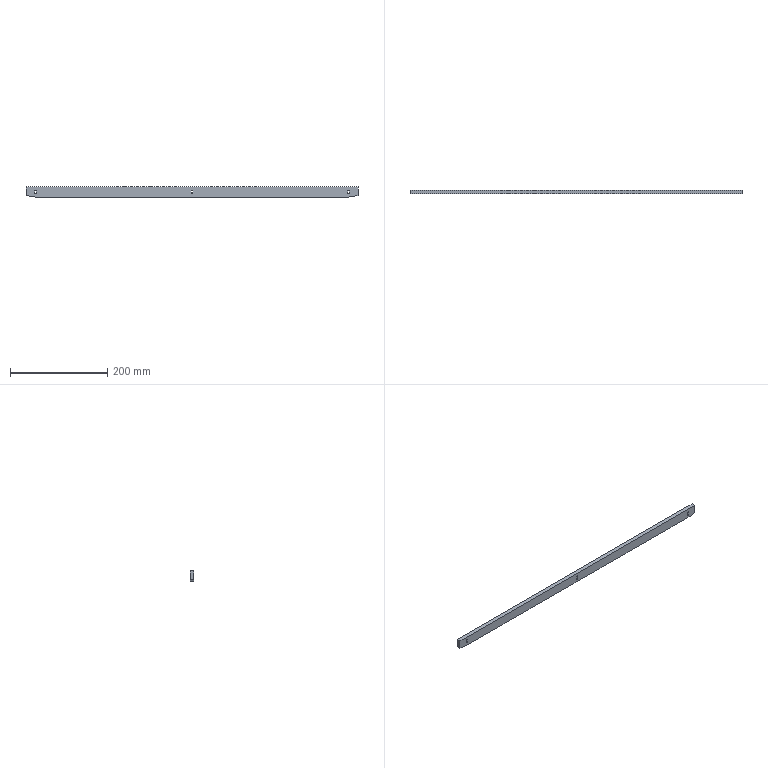Component | SolidWorks | SL010-RightStreamline-1-1_SL010-LXFB-010202-003-1-1 | 1 solid | 20 faces | box 683 x 8 x 21 mm | volume 113687 mm3 | plane 14 | cylinder 6 | commonest cylinder face diameters 3.2 x6 | material S45C
build123d program:
from build123d import *

# Parameters (mm, degrees)
SKETCH1_W           = 683
SKETCH1_H           = 21
BOSS_EXTRUDE1_DEPTH = 8
CUT_EXTRUDE1_DEPTH  = 342.755
CHAMFER1_SIZE       = 3
CHAMFER1_SIZE2      = 20
CHAMFER2_SIZE       = 20
CHAMFER2_SIZE2      = 3


with BuildPart() as part:
    # Sketch1 → Boss-Extrude1 (new body)
    with BuildSketch(Plane.XY):
        Rectangle(SKETCH1_W, SKETCH1_H)
    extrude(amount=BOSS_EXTRUDE1_DEPTH)

    # Sketch2 → Cut-Extrude1 (cut, through all)
    with BuildSketch(Plane.XY.offset(8)):
        with BuildLine():
            Line((-319.9, 2.5), (-319.9, -2.5))
            ThreePointArc((-319.9, -2.5), (-321.5, -4.1), (-323.1, -2.5))
            Line((-323.1, -2.5), (-323.1, 2.5))
            ThreePointArc((-323.1, 2.5), (-321.5, 4.1), (-319.9, 2.5))
        make_face()
        with BuildLine():
            Line((1.6, 2.5), (1.6, -2.5))
            ThreePointArc((1.6, -2.5), (0, -4.1), (-1.6, -2.5))
            Line((-1.6, -2.5), (-1.6, 2.5))
            ThreePointArc((-1.6, 2.5), (0, 4.1), (1.6, 2.5))
        make_face()
        with BuildLine():
            Line((323.1, 2.5), (323.1, -2.5))
            ThreePointArc((323.1, -2.5), (321.5, -4.1), (319.9, -2.5))
            Line((319.9, -2.5), (319.9, 2.5))
            ThreePointArc((319.9, 2.5), (321.5, 4.1), (323.1, 2.5))
        make_face()
    extrude(amount=-CUT_EXTRUDE1_DEPTH, mode=Mode.SUBTRACT)

    # Chamfer1
    chamfer1_edges = [part.edges().sort_by_distance(p)[0] for p in [
        (341.5, 10.5, 4),
    ]]
    chamfer1_side = [part.faces().sort_by_distance(p)[0] for p in [
        (341.5, 0, 4),
    ]]
    chamfer(chamfer1_edges, length=CHAMFER1_SIZE, length2=CHAMFER1_SIZE2, reference=chamfer1_side[0])

    # Chamfer2
    chamfer2_edges = [part.edges().sort_by_distance(p)[0] for p in [
        (-341.5, 10.5, 4),
    ]]
    chamfer2_side = [part.faces().sort_by_distance(p)[0] for p in [
        (-10, 10.5, 4),
    ]]
    chamfer(chamfer2_edges, length=CHAMFER2_SIZE, length2=CHAMFER2_SIZE2, reference=chamfer2_side[0])


solid = part.part

# Placed as in the assembly
solid = solid.moved(Location((633.5, -109.904, -326.535), (-90, 0, 0)))
STEP:
#1=CARTESIAN_POINT('',(38.386,-4.327,-12.442));
#2=VERTEX_POINT('',#1);
#3=CARTESIAN_POINT('',(38.386,-4.327,-13.151));
#4=VERTEX_POINT('',#3);
#5=CARTESIAN_POINT('',(38.386,-4.327,-13.269));
#6=DIRECTION('',(-0.,0.,-1.));
#7=VECTOR('',#6,39.37);
#8=LINE('',#5,#7);
#9=EDGE_CURVE('',#2,#4,#8,.T.);
#10=ORIENTED_EDGE('',*,*,#9,.T.);
#11=CARTESIAN_POINT('',(38.386,-4.012,-13.151));
#12=VERTEX_POINT('',#11);
#13=CARTESIAN_POINT('',(38.386,-4.012,-13.151));
#14=DIRECTION('',(-0.,1.,-0.));
#15=VECTOR('',#14,39.37);
#16=LINE('',#13,#15);
#17=EDGE_CURVE('',#4,#12,#16,.T.);
#18=ORIENTED_EDGE('',*,*,#17,.T.);
#19=CARTESIAN_POINT('',(38.386,-4.012,-12.442));
#20=VERTEX_POINT('',#19);
#21=CARTESIAN_POINT('',(38.386,-4.012,-13.269));
#22=DIRECTION('',(-0.,0.,-1.));
#23=VECTOR('',#22,39.37);
#24=LINE('',#21,#23);
#25=EDGE_CURVE('',#20,#12,#24,.T.);
#26=ORIENTED_EDGE('',*,*,#25,.F.);
#27=CARTESIAN_POINT('',(38.386,-4.012,-12.442));
#28=DIRECTION('',(0.,-1.,0.));
#29=VECTOR('',#28,39.37);
#30=LINE('',#27,#29);
#31=EDGE_CURVE('',#20,#2,#30,.T.);
#32=ORIENTED_EDGE('',*,*,#31,.T.);
#33=EDGE_LOOP('',(#10,#18,#26,#32));
#34=FACE_OUTER_BOUND('',#33,.T.);
#35=CARTESIAN_POINT('',(38.386,-4.012,-13.269));
#36=DIRECTION('',(-1.,-0.,-0.));
#37=DIRECTION('',(-0.,1.,-0.));
#38=AXIS2_PLACEMENT_3D('',#35,#36,#37);
#39=PLANE('',#38);
#40=ADVANCED_FACE('',(#34),#39,.F.);
#41=CARTESIAN_POINT('',(37.598,-4.327,-13.269));
#42=VERTEX_POINT('',#41);
#43=CARTESIAN_POINT('',(12.283,-4.327,-13.269));
#44=VERTEX_POINT('',#43);
#45=CARTESIAN_POINT('',(11.496,-4.327,-13.269));
#46=DIRECTION('',(-1.,0.,-0.));
#47=VECTOR('',#46,39.37);
#48=LINE('',#45,#47);
#49=EDGE_CURVE('',#42,#44,#48,.T.);
#50=ORIENTED_EDGE('',*,*,#49,.T.);
#51=CARTESIAN_POINT('',(12.283,-4.012,-13.269));
#52=VERTEX_POINT('',#51);
#53=CARTESIAN_POINT('',(12.283,-4.012,-13.269));
#54=DIRECTION('',(-0.,1.,-0.));
#55=VECTOR('',#54,39.37);
#56=LINE('',#53,#55);
#57=EDGE_CURVE('',#44,#52,#56,.T.);
#58=ORIENTED_EDGE('',*,*,#57,.T.);
#59=CARTESIAN_POINT('',(37.598,-4.012,-13.269));
#60=VERTEX_POINT('',#59);
#61=CARTESIAN_POINT('',(11.496,-4.012,-13.269));
#62=DIRECTION('',(-1.,0.,-0.));
#63=VECTOR('',#62,39.37);
#64=LINE('',#61,#63);
#65=EDGE_CURVE('',#60,#52,#64,.T.);
#66=ORIENTED_EDGE('',*,*,#65,.F.);
#67=CARTESIAN_POINT('',(37.598,-4.012,-13.269));
#68=DIRECTION('',(0.,-1.,0.));
#69=VECTOR('',#68,39.37);
#70=LINE('',#67,#69);
#71=EDGE_CURVE('',#60,#42,#70,.T.);
#72=ORIENTED_EDGE('',*,*,#71,.T.);
#73=EDGE_LOOP('',(#50,#58,#66,#72));
#74=FACE_OUTER_BOUND('',#73,.T.);
#75=CARTESIAN_POINT('',(11.496,-4.012,-13.269));
#76=DIRECTION('',(0.,0.,1.));
#77=DIRECTION('',(0.,-1.,0.));
#78=AXIS2_PLACEMENT_3D('',#75,#76,#77);
#79=PLANE('',#78);
#80=ADVANCED_FACE('',(#74),#79,.F.);
#81=CARTESIAN_POINT('',(11.496,-4.012,-13.151));
#82=VERTEX_POINT('',#81);
#83=CARTESIAN_POINT('',(11.496,-4.012,-12.442));
#84=VERTEX_POINT('',#83);
#85=CARTESIAN_POINT('',(11.496,-4.012,-13.269));
#86=DIRECTION('',(0.,-0.,1.));
#87=VECTOR('',#86,39.37);
#88=LINE('',#85,#87);
#89=EDGE_CURVE('',#82,#84,#88,.T.);
#90=ORIENTED_EDGE('',*,*,#89,.F.);
#91=CARTESIAN_POINT('',(11.496,-4.327,-13.151));
#92=VERTEX_POINT('',#91);
#93=CARTESIAN_POINT('',(11.496,-4.012,-13.151));
#94=DIRECTION('',(0.,-1.,0.));
#95=VECTOR('',#94,39.37);
#96=LINE('',#93,#95);
#97=EDGE_CURVE('',#82,#92,#96,.T.);
#98=ORIENTED_EDGE('',*,*,#97,.T.);
#99=CARTESIAN_POINT('',(11.496,-4.327,-12.442));
#100=VERTEX_POINT('',#99);
#101=CARTESIAN_POINT('',(11.496,-4.327,-13.269));
#102=DIRECTION('',(0.,-0.,1.));
#103=VECTOR('',#102,39.37);
#104=LINE('',#101,#103);
#105=EDGE_CURVE('',#92,#100,#104,.T.);
#106=ORIENTED_EDGE('',*,*,#105,.T.);
#107=CARTESIAN_POINT('',(11.496,-4.012,-12.442));
#108=DIRECTION('',(0.,-1.,0.));
#109=VECTOR('',#108,39.37);
#110=LINE('',#107,#109);
#111=EDGE_CURVE('',#84,#100,#110,.T.);
#112=ORIENTED_EDGE('',*,*,#111,.F.);
#113=EDGE_LOOP('',(#90,#98,#106,#112));
#114=FACE_OUTER_BOUND('',#113,.T.);
#115=CARTESIAN_POINT('',(11.496,-4.012,-13.269));
#116=DIRECTION('',(1.,0.,0.));
#117=DIRECTION('',(0.,-1.,0.));
#118=AXIS2_PLACEMENT_3D('',#115,#116,#117);
#119=PLANE('',#118);
#120=ADVANCED_FACE('',(#114),#119,.F.);
#121=CARTESIAN_POINT('',(11.496,-4.327,-12.442));
#122=DIRECTION('',(1.,-0.,0.));
#123=VECTOR('',#122,39.37);
#124=LINE('',#121,#123);
#125=EDGE_CURVE('',#100,#2,#124,.T.);
#126=ORIENTED_EDGE('',*,*,#125,.T.);
#127=ORIENTED_EDGE('',*,*,#31,.F.);
#128=CARTESIAN_POINT('',(11.496,-4.012,-12.442));
#129=DIRECTION('',(1.,-0.,0.));
#130=VECTOR('',#129,39.37);
#131=LINE('',#128,#130);
#132=EDGE_CURVE('',#84,#20,#131,.T.);
#133=ORIENTED_EDGE('',*,*,#132,.F.);
#134=ORIENTED_EDGE('',*,*,#111,.T.);
#135=EDGE_LOOP('',(#126,#127,#133,#134));
#136=FACE_OUTER_BOUND('',#135,.T.);
#137=CARTESIAN_POINT('',(11.496,-4.012,-12.442));
#138=DIRECTION('',(-0.,-0.,-1.));
#139=DIRECTION('',(-0.,1.,-0.));
#140=AXIS2_PLACEMENT_3D('',#137,#138,#139);
#141=PLANE('',#140);
#142=ADVANCED_FACE('',(#136),#141,.F.);
#143=CARTESIAN_POINT('',(37.661,-4.012,-12.954));
#144=VERTEX_POINT('',#143);
#145=CARTESIAN_POINT('',(37.535,-4.012,-12.954));
#146=VERTEX_POINT('',#145);
#147=CARTESIAN_POINT('',(37.598,-4.012,-12.954));
#148=DIRECTION('',(-0.,1.,-0.));
#149=DIRECTION('',(1.,0.,0.));
#150=AXIS2_PLACEMENT_3D('',#147,#148,#149);
#151=CIRCLE('',#150,0.06299);
#152=EDGE_CURVE('',#144,#146,#151,.T.);
#153=ORIENTED_EDGE('',*,*,#152,.F.);
#154=CARTESIAN_POINT('',(37.661,-4.012,-12.757));
#155=VERTEX_POINT('',#154);
#156=CARTESIAN_POINT('',(37.661,-4.012,-12.954));
#157=DIRECTION('',(-0.,0.,-1.));
#158=VECTOR('',#157,39.37);
#159=LINE('',#156,#158);
#160=EDGE_CURVE('',#155,#144,#159,.T.);
#161=ORIENTED_EDGE('',*,*,#160,.F.);
#162=CARTESIAN_POINT('',(37.535,-4.012,-12.757));
#163=VERTEX_POINT('',#162);
#164=CARTESIAN_POINT('',(37.598,-4.012,-12.757));
#165=DIRECTION('',(-0.,1.,-0.));
#166=DIRECTION('',(1.,0.,0.));
#167=AXIS2_PLACEMENT_3D('',#164,#165,#166);
#168=CIRCLE('',#167,0.06299);
#169=EDGE_CURVE('',#163,#155,#168,.T.);
#170=ORIENTED_EDGE('',*,*,#169,.F.);
#171=CARTESIAN_POINT('',(37.535,-4.012,-12.954));
#172=DIRECTION('',(0.,-0.,1.));
#173=VECTOR('',#172,39.37);
#174=LINE('',#171,#173);
#175=EDGE_CURVE('',#146,#163,#174,.T.);
#176=ORIENTED_EDGE('',*,*,#175,.F.);
#177=EDGE_LOOP('',(#153,#161,#170,#176));
#178=FACE_BOUND('',#177,.T.);
#179=CARTESIAN_POINT('',(25.004,-4.012,-12.954));
#180=VERTEX_POINT('',#179);
#181=CARTESIAN_POINT('',(24.878,-4.012,-12.954));
#182=VERTEX_POINT('',#181);
#183=CARTESIAN_POINT('',(24.941,-4.012,-12.954));
#184=DIRECTION('',(-0.,1.,-0.));
#185=DIRECTION('',(1.,0.,0.));
#186=AXIS2_PLACEMENT_3D('',#183,#184,#185);
#187=CIRCLE('',#186,0.06299);
#188=EDGE_CURVE('',#180,#182,#187,.T.);
#189=ORIENTED_EDGE('',*,*,#188,.F.);
#190=CARTESIAN_POINT('',(25.004,-4.012,-12.757));
#191=VERTEX_POINT('',#190);
#192=CARTESIAN_POINT('',(25.004,-4.012,-12.954));
#193=DIRECTION('',(-0.,0.,-1.));
#194=VECTOR('',#193,39.37);
#195=LINE('',#192,#194);
#196=EDGE_CURVE('',#191,#180,#195,.T.);
#197=ORIENTED_EDGE('',*,*,#196,.F.);
#198=CARTESIAN_POINT('',(24.878,-4.012,-12.757));
#199=VERTEX_POINT('',#198);
#200=CARTESIAN_POINT('',(24.941,-4.012,-12.757));
#201=DIRECTION('',(-0.,1.,-0.));
#202=DIRECTION('',(1.,0.,0.));
#203=AXIS2_PLACEMENT_3D('',#200,#201,#202);
#204=CIRCLE('',#203,0.06299);
#205=EDGE_CURVE('',#199,#191,#204,.T.);
#206=ORIENTED_EDGE('',*,*,#205,.F.);
#207=CARTESIAN_POINT('',(24.878,-4.012,-12.954));
#208=DIRECTION('',(0.,-0.,1.));
#209=VECTOR('',#208,39.37);
#210=LINE('',#207,#209);
#211=EDGE_CURVE('',#182,#199,#210,.T.);
#212=ORIENTED_EDGE('',*,*,#211,.F.);
#213=EDGE_LOOP('',(#189,#197,#206,#212));
#214=FACE_BOUND('',#213,.T.);
#215=CARTESIAN_POINT('',(12.346,-4.012,-12.954));
#216=VERTEX_POINT('',#215);
#217=CARTESIAN_POINT('',(12.22,-4.012,-12.954));
#218=VERTEX_POINT('',#217);
#219=CARTESIAN_POINT('',(12.283,-4.012,-12.954));
#220=DIRECTION('',(-0.,1.,-0.));
#221=DIRECTION('',(1.,0.,0.));
#222=AXIS2_PLACEMENT_3D('',#219,#220,#221);
#223=CIRCLE('',#222,0.06299);
#224=EDGE_CURVE('',#216,#218,#223,.T.);
#225=ORIENTED_EDGE('',*,*,#224,.F.);
#226=CARTESIAN_POINT('',(12.346,-4.012,-12.757));
#227=VERTEX_POINT('',#226);
#228=CARTESIAN_POINT('',(12.346,-4.012,-12.954));
#229=DIRECTION('',(-0.,0.,-1.));
#230=VECTOR('',#229,39.37);
#231=LINE('',#228,#230);
#232=EDGE_CURVE('',#227,#216,#231,.T.);
#233=ORIENTED_EDGE('',*,*,#232,.F.);
#234=CARTESIAN_POINT('',(12.22,-4.012,-12.757));
#235=VERTEX_POINT('',#234);
#236=CARTESIAN_POINT('',(12.283,-4.012,-12.757));
#237=DIRECTION('',(-0.,1.,-0.));
#238=DIRECTION('',(1.,0.,0.));
#239=AXIS2_PLACEMENT_3D('',#236,#237,#238);
#240=CIRCLE('',#239,0.06299);
#241=EDGE_CURVE('',#235,#227,#240,.T.);
#242=ORIENTED_EDGE('',*,*,#241,.F.);
#243=CARTESIAN_POINT('',(12.22,-4.012,-12.954));
#244=DIRECTION('',(0.,-0.,1.));
#245=VECTOR('',#244,39.37);
#246=LINE('',#243,#245);
#247=EDGE_CURVE('',#218,#235,#246,.T.);
#248=ORIENTED_EDGE('',*,*,#247,.F.);
#249=EDGE_LOOP('',(#225,#233,#242,#248));
#250=FACE_BOUND('',#249,.T.);
#251=ORIENTED_EDGE('',*,*,#65,.T.);
#252=CARTESIAN_POINT('',(24.602,-4.012,-15.117));
#253=DIRECTION('',(-0.9889,0.,0.1483));
#254=VECTOR('',#253,39.37);
#255=LINE('',#252,#254);
#256=EDGE_CURVE('',#52,#82,#255,.T.);
#257=ORIENTED_EDGE('',*,*,#256,.T.);
#258=ORIENTED_EDGE('',*,*,#89,.T.);
#259=ORIENTED_EDGE('',*,*,#132,.T.);
#260=ORIENTED_EDGE('',*,*,#25,.T.);
#261=CARTESIAN_POINT('',(25.28,-4.012,-15.117));
#262=DIRECTION('',(-0.9889,0.,-0.1483));
#263=VECTOR('',#262,39.37);
#264=LINE('',#261,#263);
#265=EDGE_CURVE('',#12,#60,#264,.T.);
#266=ORIENTED_EDGE('',*,*,#265,.T.);
#267=EDGE_LOOP('',(#251,#257,#258,#259,#260,#266));
#268=FACE_OUTER_BOUND('',#267,.T.);
#269=CARTESIAN_POINT('',(24.941,-4.012,-12.856));
#270=DIRECTION('',(0.,1.,-0.));
#271=DIRECTION('',(1.,-0.,0.));
#272=AXIS2_PLACEMENT_3D('',#269,#270,#271);
#273=PLANE('',#272);
#274=ADVANCED_FACE('',(#178,#214,#250,#268),#273,.T.);
#275=CARTESIAN_POINT('',(37.661,-4.327,-12.757));
#276=VERTEX_POINT('',#275);
#277=CARTESIAN_POINT('',(37.661,-4.327,-12.954));
#278=VERTEX_POINT('',#277);
#279=CARTESIAN_POINT('',(37.661,-4.327,-12.954));
#280=DIRECTION('',(-0.,0.,-1.));
#281=VECTOR('',#280,39.37);
#282=LINE('',#279,#281);
#283=EDGE_CURVE('',#276,#278,#282,.T.);
#284=ORIENTED_EDGE('',*,*,#283,.T.);
#285=CARTESIAN_POINT('',(37.535,-4.327,-12.954));
#286=VERTEX_POINT('',#285);
#287=CARTESIAN_POINT('',(37.598,-4.327,-12.954));
#288=DIRECTION('',(-0.,1.,-0.));
#289=DIRECTION('',(1.,0.,0.));
#290=AXIS2_PLACEMENT_3D('',#287,#288,#289);
#291=CIRCLE('',#290,0.06299);
#292=EDGE_CURVE('',#278,#286,#291,.T.);
#293=ORIENTED_EDGE('',*,*,#292,.T.);
#294=CARTESIAN_POINT('',(37.535,-4.327,-12.757));
#295=VERTEX_POINT('',#294);
#296=CARTESIAN_POINT('',(37.535,-4.327,-12.954));
#297=DIRECTION('',(0.,-0.,1.));
#298=VECTOR('',#297,39.37);
#299=LINE('',#296,#298);
#300=EDGE_CURVE('',#286,#295,#299,.T.);
#301=ORIENTED_EDGE('',*,*,#300,.T.);
#302=CARTESIAN_POINT('',(37.598,-4.327,-12.757));
#303=DIRECTION('',(-0.,1.,-0.));
#304=DIRECTION('',(1.,0.,0.));
#305=AXIS2_PLACEMENT_3D('',#302,#303,#304);
#306=CIRCLE('',#305,0.06299);
#307=EDGE_CURVE('',#295,#276,#306,.T.);
#308=ORIENTED_EDGE('',*,*,#307,.T.);
#309=EDGE_LOOP('',(#284,#293,#301,#308));
#310=FACE_BOUND('',#309,.T.);
#311=CARTESIAN_POINT('',(25.004,-4.327,-12.757));
#312=VERTEX_POINT('',#311);
#313=CARTESIAN_POINT('',(25.004,-4.327,-12.954));
#314=VERTEX_POINT('',#313);
#315=CARTESIAN_POINT('',(25.004,-4.327,-12.954));
#316=DIRECTION('',(-0.,0.,-1.));
#317=VECTOR('',#316,39.37);
#318=LINE('',#315,#317);
#319=EDGE_CURVE('',#312,#314,#318,.T.);
#320=ORIENTED_EDGE('',*,*,#319,.T.);
#321=CARTESIAN_POINT('',(24.878,-4.327,-12.954));
#322=VERTEX_POINT('',#321);
#323=CARTESIAN_POINT('',(24.941,-4.327,-12.954));
#324=DIRECTION('',(-0.,1.,-0.));
#325=DIRECTION('',(1.,0.,0.));
#326=AXIS2_PLACEMENT_3D('',#323,#324,#325);
#327=CIRCLE('',#326,0.06299);
#328=EDGE_CURVE('',#314,#322,#327,.T.);
#329=ORIENTED_EDGE('',*,*,#328,.T.);
#330=CARTESIAN_POINT('',(24.878,-4.327,-12.757));
#331=VERTEX_POINT('',#330);
#332=CARTESIAN_POINT('',(24.878,-4.327,-12.954));
#333=DIRECTION('',(0.,-0.,1.));
#334=VECTOR('',#333,39.37);
#335=LINE('',#332,#334);
#336=EDGE_CURVE('',#322,#331,#335,.T.);
#337=ORIENTED_EDGE('',*,*,#336,.T.);
#338=CARTESIAN_POINT('',(24.941,-4.327,-12.757));
#339=DIRECTION('',(-0.,1.,-0.));
#340=DIRECTION('',(1.,0.,0.));
#341=AXIS2_PLACEMENT_3D('',#338,#339,#340);
#342=CIRCLE('',#341,0.06299);
#343=EDGE_CURVE('',#331,#312,#342,.T.);
#344=ORIENTED_EDGE('',*,*,#343,.T.);
#345=EDGE_LOOP('',(#320,#329,#337,#344));
#346=FACE_BOUND('',#345,.T.);
#347=CARTESIAN_POINT('',(12.346,-4.327,-12.757));
#348=VERTEX_POINT('',#347);
#349=CARTESIAN_POINT('',(12.346,-4.327,-12.954));
#350=VERTEX_POINT('',#349);
#351=CARTESIAN_POINT('',(12.346,-4.327,-12.954));
#352=DIRECTION('',(-0.,0.,-1.));
#353=VECTOR('',#352,39.37);
#354=LINE('',#351,#353);
#355=EDGE_CURVE('',#348,#350,#354,.T.);
#356=ORIENTED_EDGE('',*,*,#355,.T.);
#357=CARTESIAN_POINT('',(12.22,-4.327,-12.954));
#358=VERTEX_POINT('',#357);
#359=CARTESIAN_POINT('',(12.283,-4.327,-12.954));
#360=DIRECTION('',(-0.,1.,-0.));
#361=DIRECTION('',(1.,0.,0.));
#362=AXIS2_PLACEMENT_3D('',#359,#360,#361);
#363=CIRCLE('',#362,0.06299);
#364=EDGE_CURVE('',#350,#358,#363,.T.);
#365=ORIENTED_EDGE('',*,*,#364,.T.);
#366=CARTESIAN_POINT('',(12.22,-4.327,-12.757));
#367=VERTEX_POINT('',#366);
#368=CARTESIAN_POINT('',(12.22,-4.327,-12.954));
#369=DIRECTION('',(0.,-0.,1.));
#370=VECTOR('',#369,39.37);
#371=LINE('',#368,#370);
#372=EDGE_CURVE('',#358,#367,#371,.T.);
#373=ORIENTED_EDGE('',*,*,#372,.T.);
#374=CARTESIAN_POINT('',(12.283,-4.327,-12.757));
#375=DIRECTION('',(-0.,1.,-0.));
#376=DIRECTION('',(1.,0.,0.));
#377=AXIS2_PLACEMENT_3D('',#374,#375,#376);
#378=CIRCLE('',#377,0.06299);
#379=EDGE_CURVE('',#367,#348,#378,.T.);
#380=ORIENTED_EDGE('',*,*,#379,.T.);
#381=EDGE_LOOP('',(#356,#365,#373,#380));
#382=FACE_BOUND('',#381,.T.);
#383=ORIENTED_EDGE('',*,*,#105,.F.);
#384=CARTESIAN_POINT('',(11.496,-4.327,-13.151));
#385=DIRECTION('',(0.9889,-0.,-0.1483));
#386=VECTOR('',#385,39.37);
#387=LINE('',#384,#386);
#388=EDGE_CURVE('',#92,#44,#387,.T.);
#389=ORIENTED_EDGE('',*,*,#388,.T.);
#390=ORIENTED_EDGE('',*,*,#49,.F.);
#391=CARTESIAN_POINT('',(37.598,-4.327,-13.269));
#392=DIRECTION('',(0.9889,-0.,0.1483));
#393=VECTOR('',#392,39.37);
#394=LINE('',#391,#393);
#395=EDGE_CURVE('',#42,#4,#394,.T.);
#396=ORIENTED_EDGE('',*,*,#395,.T.);
#397=ORIENTED_EDGE('',*,*,#9,.F.);
#398=ORIENTED_EDGE('',*,*,#125,.F.);
#399=EDGE_LOOP('',(#383,#389,#390,#396,#397,#398));
#400=FACE_OUTER_BOUND('',#399,.T.);
#401=CARTESIAN_POINT('',(24.941,-4.327,-12.856));
#402=DIRECTION('',(0.,1.,-0.));
#403=DIRECTION('',(1.,-0.,0.));
#404=AXIS2_PLACEMENT_3D('',#401,#402,#403);
#405=PLANE('',#404);
#406=ADVANCED_FACE('',(#310,#346,#382,#400),#405,.F.);
#407=ORIENTED_EDGE('',*,*,#224,.T.);
#408=CARTESIAN_POINT('',(12.22,-4.327,-12.954));
#409=DIRECTION('',(-0.,1.,-0.));
#410=VECTOR('',#409,39.37);
#411=LINE('',#408,#410);
#412=EDGE_CURVE('',#358,#218,#411,.T.);
#413=ORIENTED_EDGE('',*,*,#412,.F.);
#414=ORIENTED_EDGE('',*,*,#364,.F.);
#415=CARTESIAN_POINT('',(12.346,-4.327,-12.954));
#416=DIRECTION('',(-0.,1.,-0.));
#417=VECTOR('',#416,39.37);
#418=LINE('',#415,#417);
#419=EDGE_CURVE('',#350,#216,#418,.T.);
#420=ORIENTED_EDGE('',*,*,#419,.T.);
#421=EDGE_LOOP('',(#407,#413,#414,#420));
#422=FACE_OUTER_BOUND('',#421,.T.);
#423=CARTESIAN_POINT('',(12.283,-4.327,-12.954));
#424=DIRECTION('',(-0.,1.,-0.));
#425=DIRECTION('',(1.,0.,0.));
#426=AXIS2_PLACEMENT_3D('',#423,#424,#425);
#427=CYLINDRICAL_SURFACE('',#426,0.06299);
#428=ADVANCED_FACE('',(#422),#427,.F.);
#429=ORIENTED_EDGE('',*,*,#232,.T.);
#430=ORIENTED_EDGE('',*,*,#419,.F.);
#431=ORIENTED_EDGE('',*,*,#355,.F.);
#432=CARTESIAN_POINT('',(12.346,-4.327,-12.757));
#433=DIRECTION('',(-0.,1.,-0.));
#434=VECTOR('',#433,39.37);
#435=LINE('',#432,#434);
#436=EDGE_CURVE('',#348,#227,#435,.T.);
#437=ORIENTED_EDGE('',*,*,#436,.T.);
#438=EDGE_LOOP('',(#429,#430,#431,#437));
#439=FACE_OUTER_BOUND('',#438,.T.);
#440=CARTESIAN_POINT('',(12.346,-4.327,-12.954));
#441=DIRECTION('',(1.,0.,0.));
#442=DIRECTION('',(0.,-1.,0.));
#443=AXIS2_PLACEMENT_3D('',#440,#441,#442);
#444=PLANE('',#443);
#445=ADVANCED_FACE('',(#439),#444,.F.);
#446=ORIENTED_EDGE('',*,*,#241,.T.);
#447=ORIENTED_EDGE('',*,*,#436,.F.);
#448=ORIENTED_EDGE('',*,*,#379,.F.);
#449=CARTESIAN_POINT('',(12.22,-4.327,-12.757));
#450=DIRECTION('',(-0.,1.,-0.));
#451=VECTOR('',#450,39.37);
#452=LINE('',#449,#451);
#453=EDGE_CURVE('',#367,#235,#452,.T.);
#454=ORIENTED_EDGE('',*,*,#453,.T.);
#455=EDGE_LOOP('',(#446,#447,#448,#454));
#456=FACE_OUTER_BOUND('',#455,.T.);
#457=CARTESIAN_POINT('',(12.283,-4.327,-12.757));
#458=DIRECTION('',(-0.,1.,-0.));
#459=DIRECTION('',(1.,0.,0.));
#460=AXIS2_PLACEMENT_3D('',#457,#458,#459);
#461=CYLINDRICAL_SURFACE('',#460,0.06299);
#462=ADVANCED_FACE('',(#456),#461,.F.);
#463=ORIENTED_EDGE('',*,*,#247,.T.);
#464=ORIENTED_EDGE('',*,*,#453,.F.);
#465=ORIENTED_EDGE('',*,*,#372,.F.);
#466=ORIENTED_EDGE('',*,*,#412,.T.);
#467=EDGE_LOOP('',(#463,#464,#465,#466));
#468=FACE_OUTER_BOUND('',#467,.T.);
#469=CARTESIAN_POINT('',(12.22,-4.327,-12.954));
#470=DIRECTION('',(-1.,-0.,-0.));
#471=DIRECTION('',(-0.,1.,-0.));
#472=AXIS2_PLACEMENT_3D('',#469,#470,#471);
#473=PLANE('',#472);
#474=ADVANCED_FACE('',(#468),#473,.F.);
#475=ORIENTED_EDGE('',*,*,#188,.T.);
#476=CARTESIAN_POINT('',(24.878,-4.327,-12.954));
#477=DIRECTION('',(-0.,1.,-0.));
#478=VECTOR('',#477,39.37);
#479=LINE('',#476,#478);
#480=EDGE_CURVE('',#322,#182,#479,.T.);
#481=ORIENTED_EDGE('',*,*,#480,.F.);
#482=ORIENTED_EDGE('',*,*,#328,.F.);
#483=CARTESIAN_POINT('',(25.004,-4.327,-12.954));
#484=DIRECTION('',(-0.,1.,-0.));
#485=VECTOR('',#484,39.37);
#486=LINE('',#483,#485);
#487=EDGE_CURVE('',#314,#180,#486,.T.);
#488=ORIENTED_EDGE('',*,*,#487,.T.);
#489=EDGE_LOOP('',(#475,#481,#482,#488));
#490=FACE_OUTER_BOUND('',#489,.T.);
#491=CARTESIAN_POINT('',(24.941,-4.327,-12.954));
#492=DIRECTION('',(-0.,1.,-0.));
#493=DIRECTION('',(1.,0.,0.));
#494=AXIS2_PLACEMENT_3D('',#491,#492,#493);
#495=CYLINDRICAL_SURFACE('',#494,0.06299);
#496=ADVANCED_FACE('',(#490),#495,.F.);
#497=ORIENTED_EDGE('',*,*,#196,.T.);
#498=ORIENTED_EDGE('',*,*,#487,.F.);
#499=ORIENTED_EDGE('',*,*,#319,.F.);
#500=CARTESIAN_POINT('',(25.004,-4.327,-12.757));
#501=DIRECTION('',(-0.,1.,-0.));
#502=VECTOR('',#501,39.37);
#503=LINE('',#500,#502);
#504=EDGE_CURVE('',#312,#191,#503,.T.);
#505=ORIENTED_EDGE('',*,*,#504,.T.);
#506=EDGE_LOOP('',(#497,#498,#499,#505));
#507=FACE_OUTER_BOUND('',#506,.T.);
#508=CARTESIAN_POINT('',(25.004,-4.327,-12.954));
#509=DIRECTION('',(1.,0.,0.));
#510=DIRECTION('',(0.,-1.,0.));
#511=AXIS2_PLACEMENT_3D('',#508,#509,#510);
#512=PLANE('',#511);
#513=ADVANCED_FACE('',(#507),#512,.F.);
#514=ORIENTED_EDGE('',*,*,#205,.T.);
#515=ORIENTED_EDGE('',*,*,#504,.F.);
#516=ORIENTED_EDGE('',*,*,#343,.F.);
#517=CARTESIAN_POINT('',(24.878,-4.327,-12.757));
#518=DIRECTION('',(-0.,1.,-0.));
#519=VECTOR('',#518,39.37);
#520=LINE('',#517,#519);
#521=EDGE_CURVE('',#331,#199,#520,.T.);
#522=ORIENTED_EDGE('',*,*,#521,.T.);
#523=EDGE_LOOP('',(#514,#515,#516,#522));
#524=FACE_OUTER_BOUND('',#523,.T.);
#525=CARTESIAN_POINT('',(24.941,-4.327,-12.757));
#526=DIRECTION('',(-0.,1.,-0.));
#527=DIRECTION('',(1.,0.,0.));
#528=AXIS2_PLACEMENT_3D('',#525,#526,#527);
#529=CYLINDRICAL_SURFACE('',#528,0.06299);
#530=ADVANCED_FACE('',(#524),#529,.F.);
#531=ORIENTED_EDGE('',*,*,#211,.T.);
#532=ORIENTED_EDGE('',*,*,#521,.F.);
#533=ORIENTED_EDGE('',*,*,#336,.F.);
#534=ORIENTED_EDGE('',*,*,#480,.T.);
#535=EDGE_LOOP('',(#531,#532,#533,#534));
#536=FACE_OUTER_BOUND('',#535,.T.);
#537=CARTESIAN_POINT('',(24.878,-4.327,-12.954));
#538=DIRECTION('',(-1.,-0.,-0.));
#539=DIRECTION('',(-0.,1.,-0.));
#540=AXIS2_PLACEMENT_3D('',#537,#538,#539);
#541=PLANE('',#540);
#542=ADVANCED_FACE('',(#536),#541,.F.);
#543=ORIENTED_EDGE('',*,*,#152,.T.);
#544=CARTESIAN_POINT('',(37.535,-4.327,-12.954));
#545=DIRECTION('',(-0.,1.,-0.));
#546=VECTOR('',#545,39.37);
#547=LINE('',#544,#546);
#548=EDGE_CURVE('',#286,#146,#547,.T.);
#549=ORIENTED_EDGE('',*,*,#548,.F.);
#550=ORIENTED_EDGE('',*,*,#292,.F.);
#551=CARTESIAN_POINT('',(37.661,-4.327,-12.954));
#552=DIRECTION('',(-0.,1.,-0.));
#553=VECTOR('',#552,39.37);
#554=LINE('',#551,#553);
#555=EDGE_CURVE('',#278,#144,#554,.T.);
#556=ORIENTED_EDGE('',*,*,#555,.T.);
#557=EDGE_LOOP('',(#543,#549,#550,#556));
#558=FACE_OUTER_BOUND('',#557,.T.);
#559=CARTESIAN_POINT('',(37.598,-4.327,-12.954));
#560=DIRECTION('',(-0.,1.,-0.));
#561=DIRECTION('',(1.,0.,0.));
#562=AXIS2_PLACEMENT_3D('',#559,#560,#561);
#563=CYLINDRICAL_SURFACE('',#562,0.06299);
#564=ADVANCED_FACE('',(#558),#563,.F.);
#565=ORIENTED_EDGE('',*,*,#160,.T.);
#566=ORIENTED_EDGE('',*,*,#555,.F.);
#567=ORIENTED_EDGE('',*,*,#283,.F.);
#568=CARTESIAN_POINT('',(37.661,-4.327,-12.757));
#569=DIRECTION('',(-0.,1.,-0.));
#570=VECTOR('',#569,39.37);
#571=LINE('',#568,#570);
#572=EDGE_CURVE('',#276,#155,#571,.T.);
#573=ORIENTED_EDGE('',*,*,#572,.T.);
#574=EDGE_LOOP('',(#565,#566,#567,#573));
#575=FACE_OUTER_BOUND('',#574,.T.);
#576=CARTESIAN_POINT('',(37.661,-4.327,-12.954));
#577=DIRECTION('',(1.,0.,0.));
#578=DIRECTION('',(0.,-1.,0.));
#579=AXIS2_PLACEMENT_3D('',#576,#577,#578);
#580=PLANE('',#579);
#581=ADVANCED_FACE('',(#575),#580,.F.);
#582=ORIENTED_EDGE('',*,*,#169,.T.);
#583=ORIENTED_EDGE('',*,*,#572,.F.);
#584=ORIENTED_EDGE('',*,*,#307,.F.);
#585=CARTESIAN_POINT('',(37.535,-4.327,-12.757));
#586=DIRECTION('',(-0.,1.,-0.));
#587=VECTOR('',#586,39.37);
#588=LINE('',#585,#587);
#589=EDGE_CURVE('',#295,#163,#588,.T.);
#590=ORIENTED_EDGE('',*,*,#589,.T.);
#591=EDGE_LOOP('',(#582,#583,#584,#590));
#592=FACE_OUTER_BOUND('',#591,.T.);
#593=CARTESIAN_POINT('',(37.598,-4.327,-12.757));
#594=DIRECTION('',(-0.,1.,-0.));
#595=DIRECTION('',(1.,0.,0.));
#596=AXIS2_PLACEMENT_3D('',#593,#594,#595);
#597=CYLINDRICAL_SURFACE('',#596,0.06299);
#598=ADVANCED_FACE('',(#592),#597,.F.);
#599=ORIENTED_EDGE('',*,*,#175,.T.);
#600=ORIENTED_EDGE('',*,*,#589,.F.);
#601=ORIENTED_EDGE('',*,*,#300,.F.);
#602=ORIENTED_EDGE('',*,*,#548,.T.);
#603=EDGE_LOOP('',(#599,#600,#601,#602));
#604=FACE_OUTER_BOUND('',#603,.T.);
#605=CARTESIAN_POINT('',(37.535,-4.327,-12.954));
#606=DIRECTION('',(-1.,-0.,-0.));
#607=DIRECTION('',(-0.,1.,-0.));
#608=AXIS2_PLACEMENT_3D('',#605,#606,#607);
#609=PLANE('',#608);
#610=ADVANCED_FACE('',(#604),#609,.F.);
#611=ORIENTED_EDGE('',*,*,#265,.F.);
#612=ORIENTED_EDGE('',*,*,#17,.F.);
#613=ORIENTED_EDGE('',*,*,#395,.F.);
#614=ORIENTED_EDGE('',*,*,#71,.F.);
#615=EDGE_LOOP('',(#611,#612,#613,#614));
#616=FACE_OUTER_BOUND('',#615,.T.);
#617=CARTESIAN_POINT('',(37.598,-4.012,-13.269));
#618=DIRECTION('',(-0.1483,0.,0.9889));
#619=DIRECTION('',(0.,-1.,0.));
#620=AXIS2_PLACEMENT_3D('',#617,#618,#619);
#621=PLANE('',#620);
#622=ADVANCED_FACE('',(#616),#621,.F.);
#623=ORIENTED_EDGE('',*,*,#256,.F.);
#624=ORIENTED_EDGE('',*,*,#57,.F.);
#625=ORIENTED_EDGE('',*,*,#388,.F.);
#626=ORIENTED_EDGE('',*,*,#97,.F.);
#627=EDGE_LOOP('',(#623,#624,#625,#626));
#628=FACE_OUTER_BOUND('',#627,.T.);
#629=CARTESIAN_POINT('',(11.496,-4.012,-13.151));
#630=DIRECTION('',(0.1483,0.,0.9889));
#631=DIRECTION('',(0.,-1.,0.));
#632=AXIS2_PLACEMENT_3D('',#629,#630,#631);
#633=PLANE('',#632);
#634=ADVANCED_FACE('',(#628),#633,.F.);
#635=CLOSED_SHELL('',(#40,#80,#120,#142,#274,#406,#428,#445,#462,#474,#496,#513,#530,#542,#564,#581,#598,#610,#622,#634));
#636=MANIFOLD_SOLID_BREP('',#635);
#637=CARTESIAN_POINT('',(0.,0.,0.));
#638=DIRECTION('',(0.,0.,1.));
#639=DIRECTION('',(1.,0.,0.));
#640=AXIS2_PLACEMENT_3D('',#637,#638,#639);
#641=(LENGTH_UNIT()NAMED_UNIT(*)SI_UNIT($,.METRE.));
#642=LENGTH_MEASURE_WITH_UNIT(LENGTH_MEASURE(0.0254),#641);
#643=DIMENSIONAL_EXPONENTS(1.,0.,0.,0.,0.,0.,0.);
#644=(CONVERSION_BASED_UNIT('',#642)LENGTH_UNIT()NAMED_UNIT(#643));
#645=UNCERTAINTY_MEASURE_WITH_UNIT(LENGTH_MEASURE(0.00001),#644,'','');
#646=(NAMED_UNIT(*)PLANE_ANGLE_UNIT()SI_UNIT($,.RADIAN.));
#647=(NAMED_UNIT(*)SI_UNIT($,.STERADIAN.)SOLID_ANGLE_UNIT());
#648=(GEOMETRIC_REPRESENTATION_CONTEXT(3)GLOBAL_UNCERTAINTY_ASSIGNED_CONTEXT((#645))GLOBAL_UNIT_ASSIGNED_CONTEXT((#644,#646,#647))REPRESENTATION_CONTEXT('',''));
#649=ADVANCED_BREP_SHAPE_REPRESENTATION('',(#636,#640),#648);
#650=COLOUR_RGB('',0.7922,0.8196,0.9333);
#651=FILL_AREA_STYLE_COLOUR('',#650);
#652=FILL_AREA_STYLE('',(#651));
#653=SURFACE_STYLE_FILL_AREA(#652);
#654=SURFACE_SIDE_STYLE('',(#653));
#655=SURFACE_STYLE_USAGE(.BOTH.,#654);
#656=PRESENTATION_STYLE_ASSIGNMENT((#655));
#657=STYLED_ITEM('',(#656),#636);
#658=(LENGTH_UNIT()NAMED_UNIT(*)SI_UNIT($,.METRE.));
#659=LENGTH_MEASURE_WITH_UNIT(LENGTH_MEASURE(0.0254),#658);
#660=DIMENSIONAL_EXPONENTS(1.,0.,0.,0.,0.,0.,0.);
#661=(CONVERSION_BASED_UNIT('',#659)LENGTH_UNIT()NAMED_UNIT(#660));
#662=UNCERTAINTY_MEASURE_WITH_UNIT(LENGTH_MEASURE(0.00001),#661,'','');
#663=(NAMED_UNIT(*)PLANE_ANGLE_UNIT()SI_UNIT($,.RADIAN.));
#664=(NAMED_UNIT(*)SI_UNIT($,.STERADIAN.)SOLID_ANGLE_UNIT());
#665=(GEOMETRIC_REPRESENTATION_CONTEXT(3)GLOBAL_UNCERTAINTY_ASSIGNED_CONTEXT((#662))GLOBAL_UNIT_ASSIGNED_CONTEXT((#661,#663,#664))REPRESENTATION_CONTEXT('',''));
#666=MECHANICAL_DESIGN_GEOMETRIC_PRESENTATION_REPRESENTATION('',(#657),#665);
#667=PRESENTATION_LAYER_ASSIGNMENT('','',(#657));